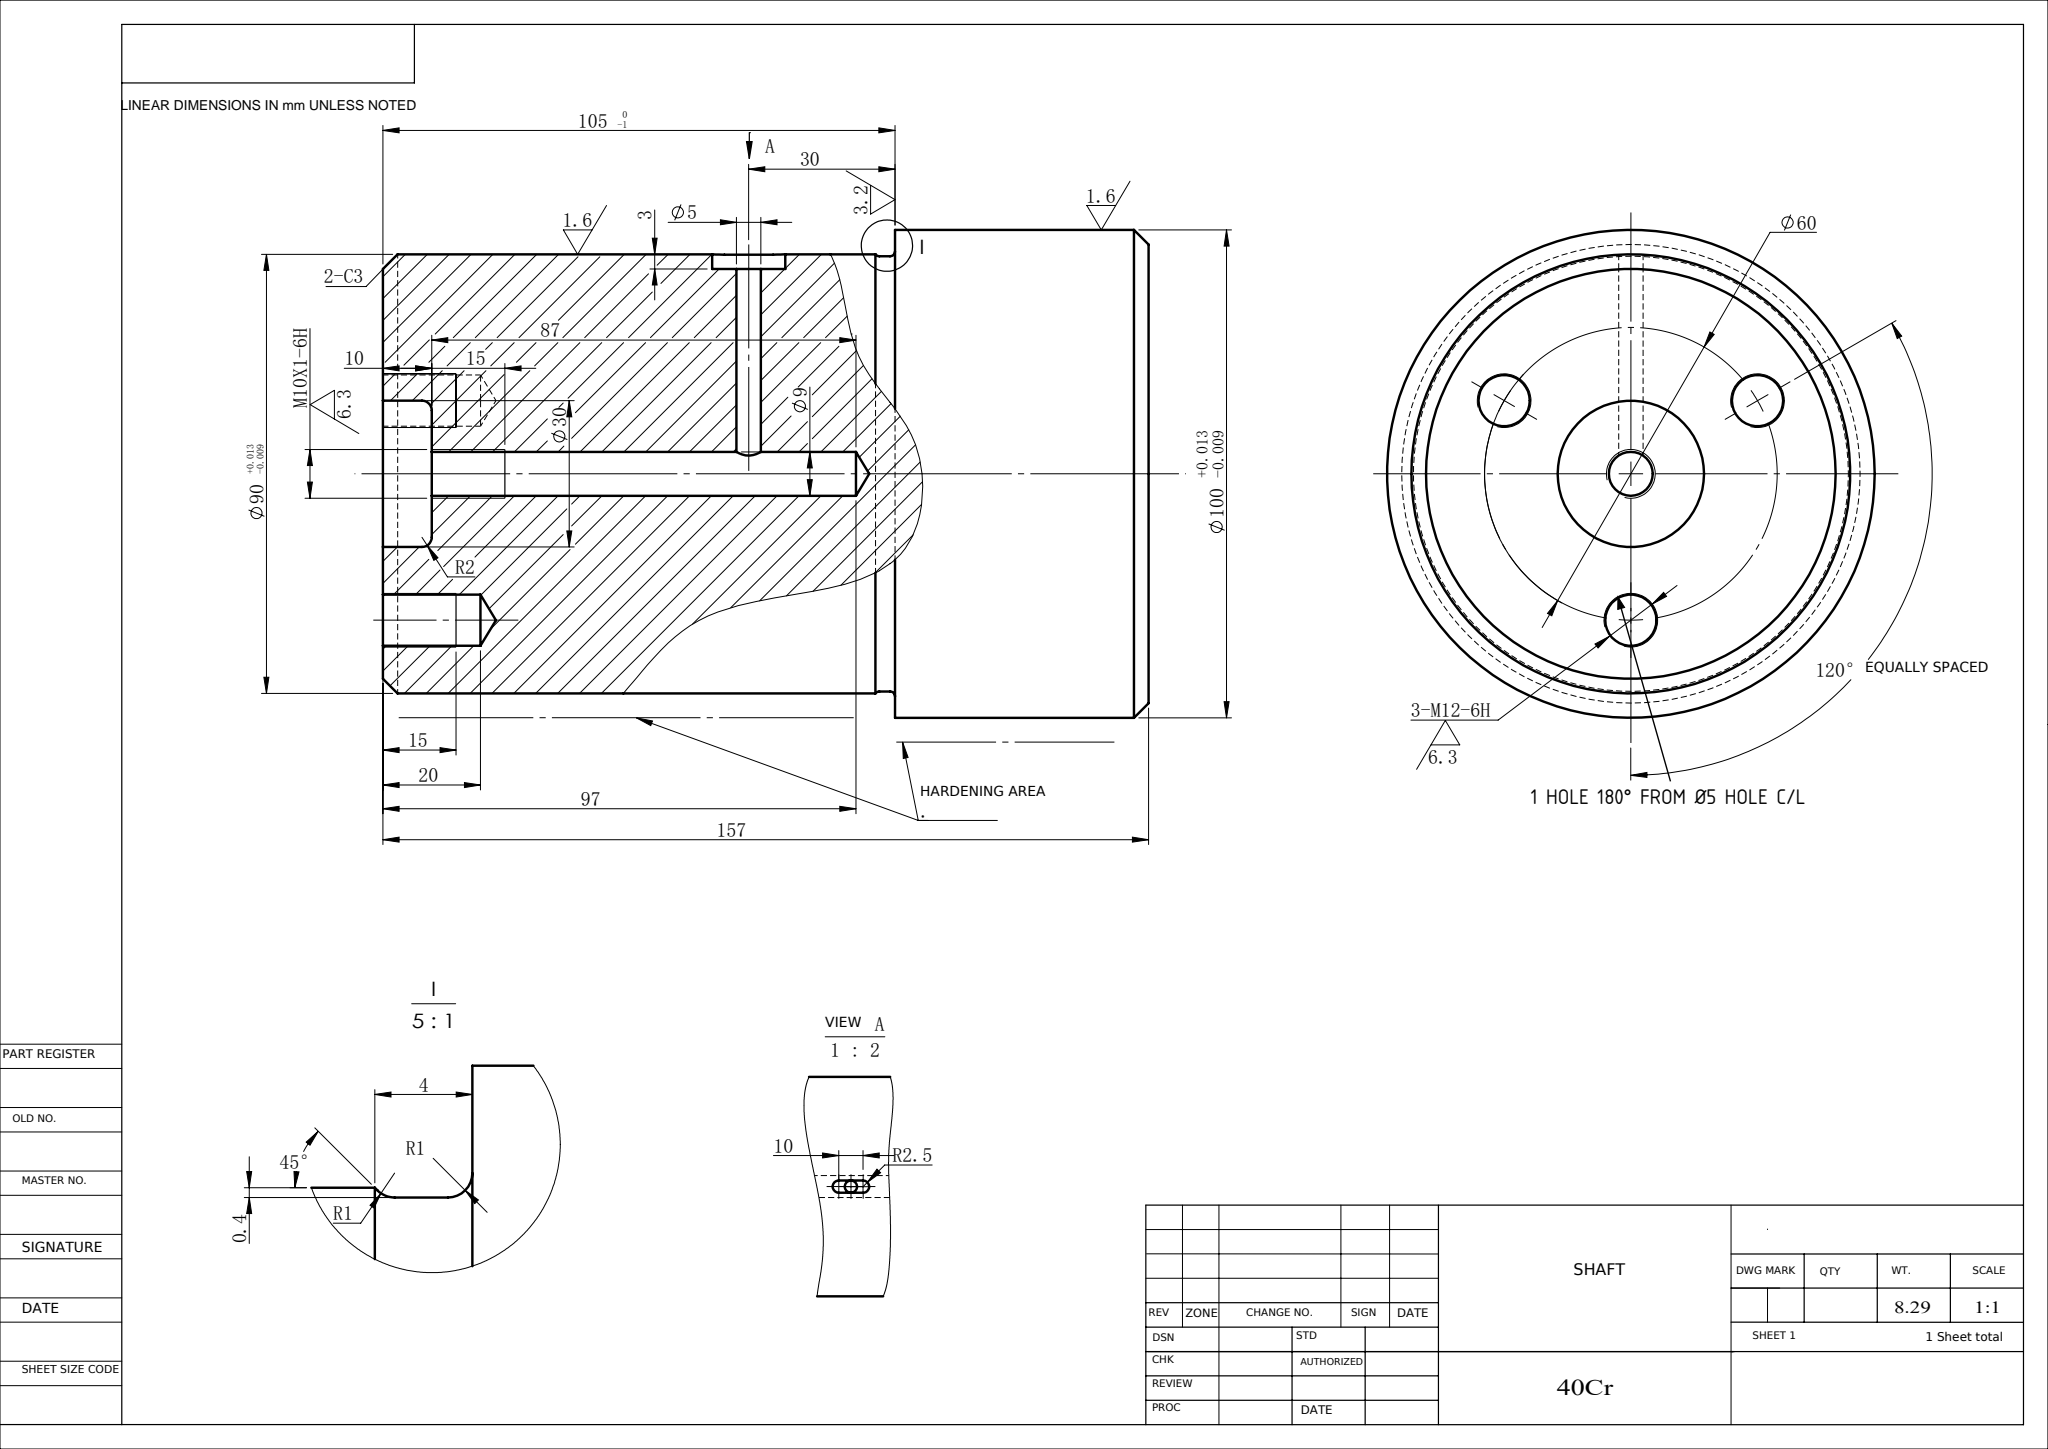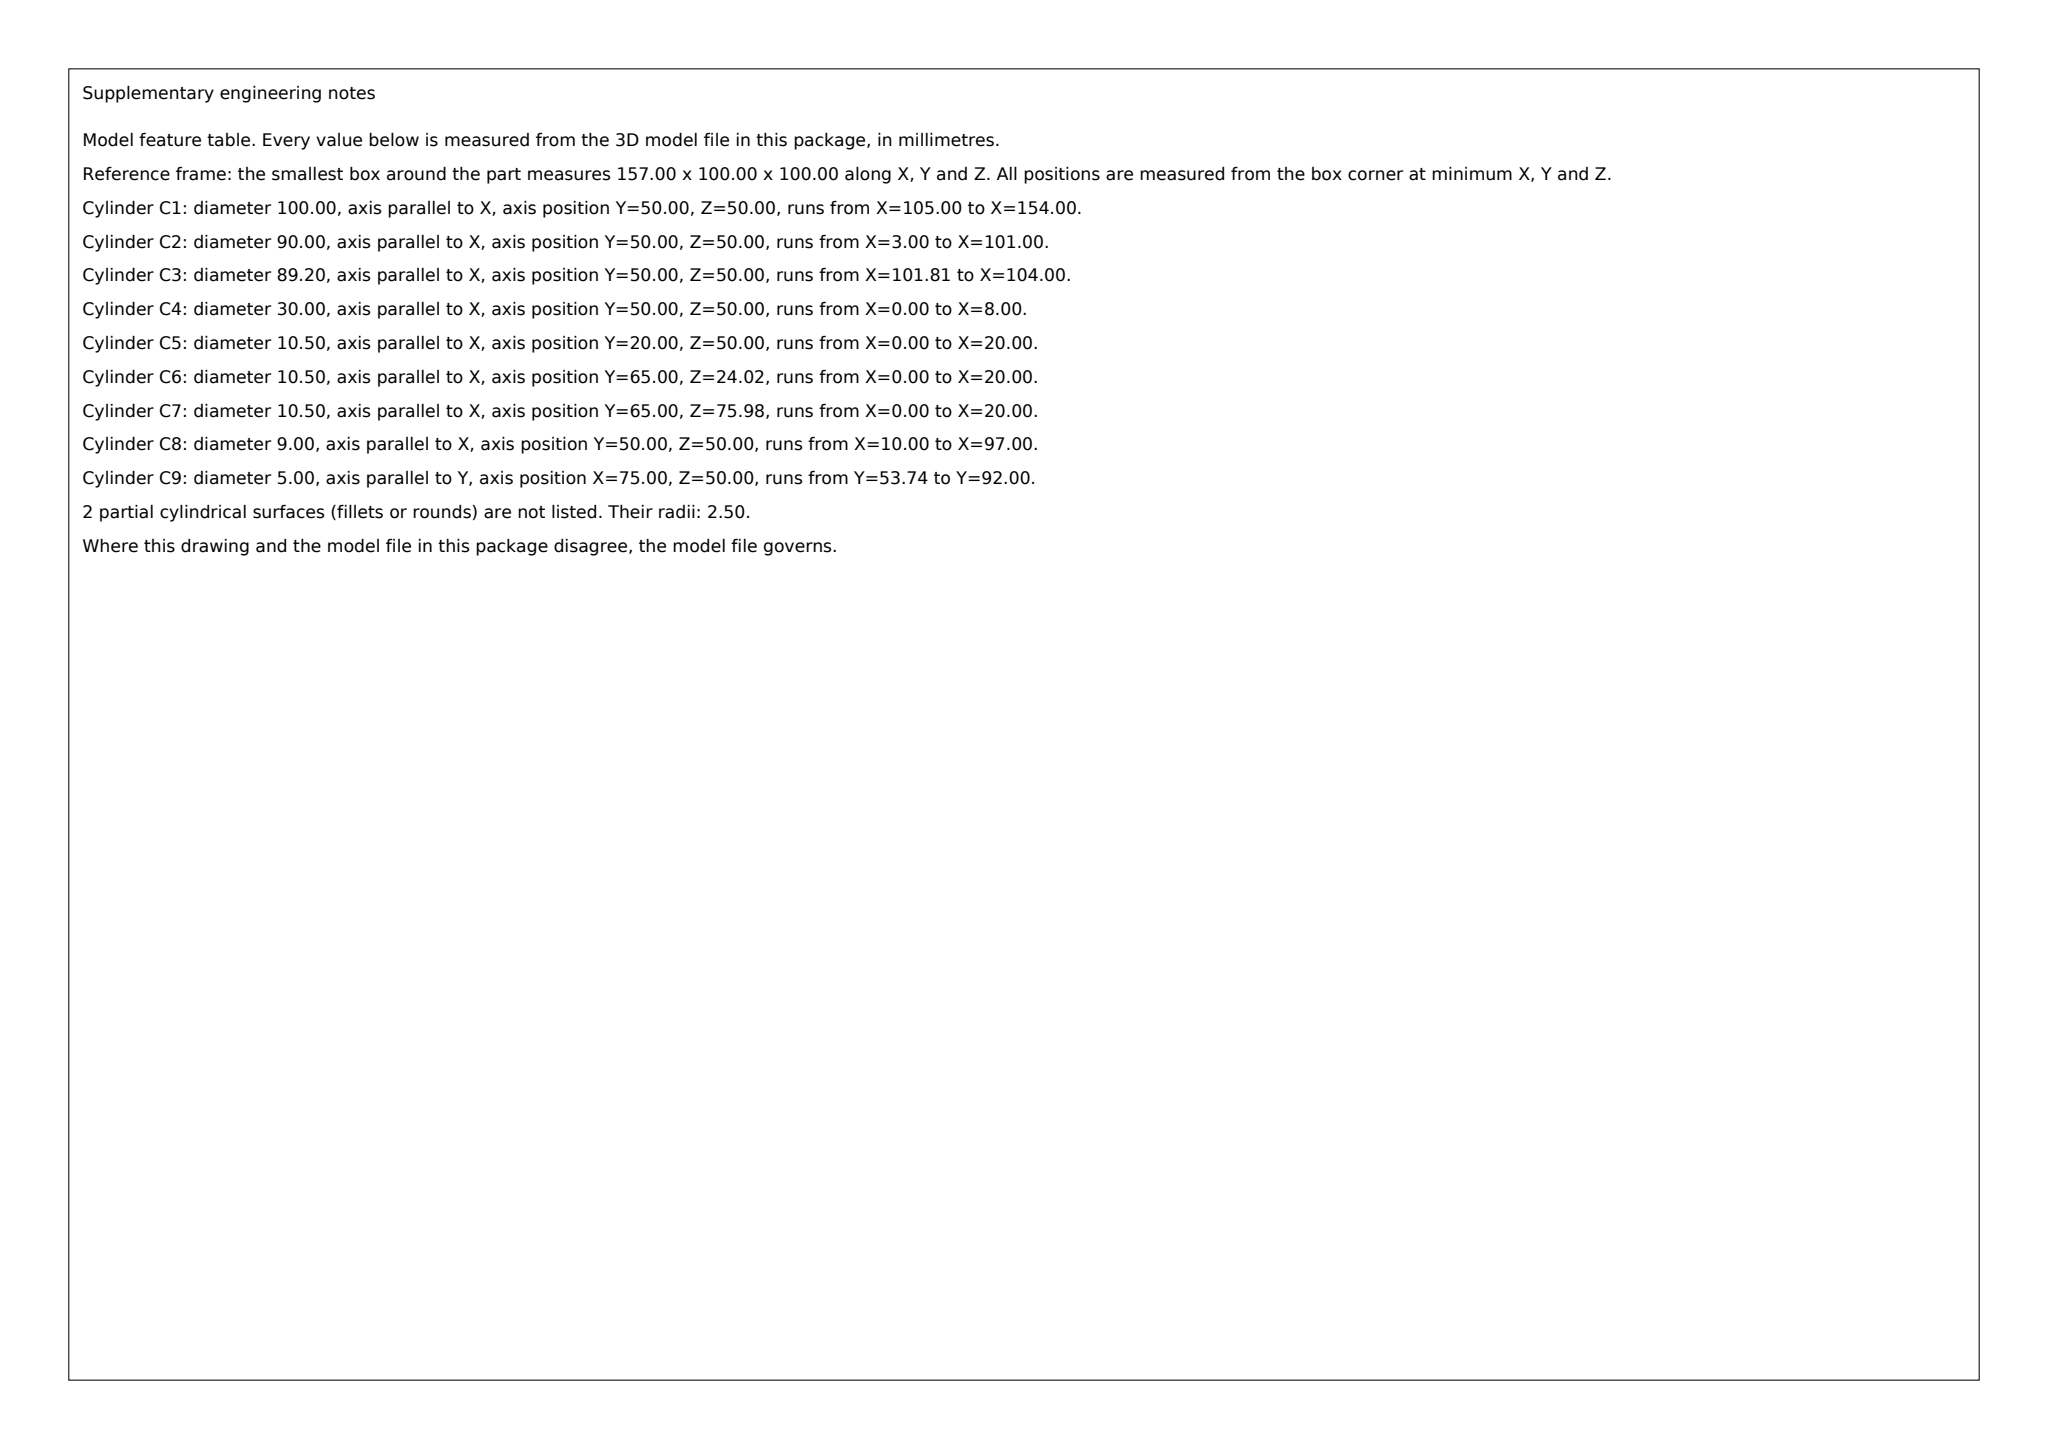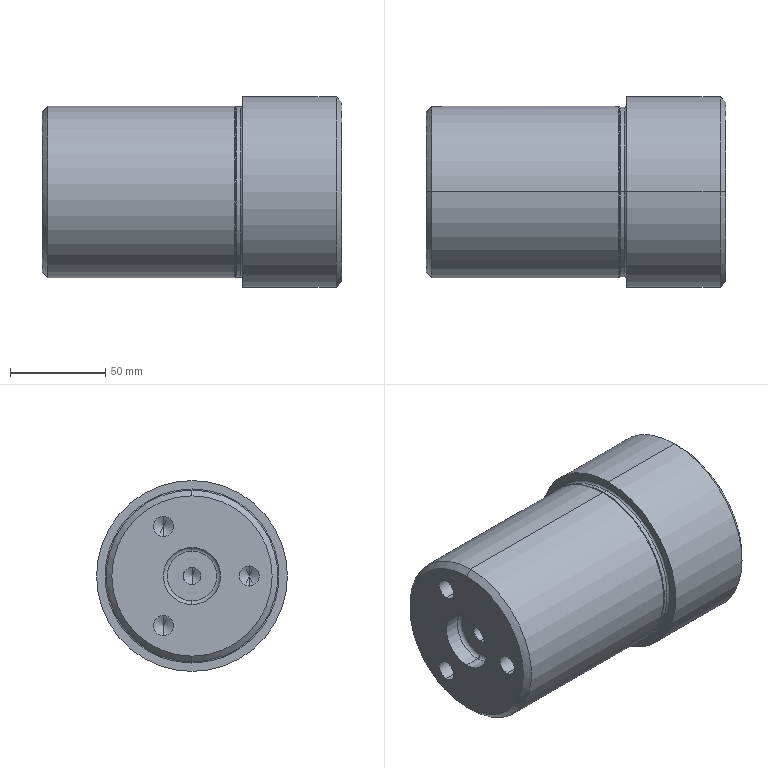Part | SolidWorks | mm | material 40Cr | 1 solid | 48 faces | box 157 x 100 x 100 mm | volume 1054399 mm3 | cylinder 20 | cone 14 | plane 8 | torus 6 | commonest cylinder face diameters 10.5 x6 5 x4 9 x2 30 x2 100 x2 89.2 x2 90 x2
Drawing notes:
3-M12-6H CLOCKING: 1 HOLE 180° FROM Ø5 CROSS HOLE C/L, OTHERS ±60° | from the solid: M12 tap drills Ø10.5 at (y,z)=(20.1,50.1),(65.1,24.1),(65.1,76.1) about axis (50.1,50.1); Ø5 cross hole axis y at z=50.1 exits +y side, so one hole lies on same C/L diametrically opposite, others at ±60° (120° equally spaced)
build123d program:
from build123d import *

# Parameters (mm, degrees)
FILLET1_R                  = 1
CHAMFER1_SIZE              = 3
SKETCH2_R                  = 15
CUT_EXTRUDE1_DEPTH         = 10
M10X1_0_TAPPED_HOLE1_D     = 9
M10X1_0_TAPPED_HOLE1_DEPTH = 87
M10X1_0_TAPPED_HOLE1_TIP   = 2.704
CUT_EXTRUDE2_DEPTH         = 3
CUT_EXTRUDE3_REACH         = 190.714
CUT_EXTRUDE3_END_RADIUS    = 4.5
SKETCH7_R                  = 2.5
FILLET2_R                  = 2
CIRPATTERN1_COUNT          = 3


with BuildPart() as part:
    # Sketch1 → Revolve1 (revolve)
    with BuildSketch(Plane.XY, mode=Mode.PRIVATE) as revolve1_sk:
        with BuildLine():
            Line((0, 0), (0, 45))
            Line((0, 45), (101, 45))
            Line((101, 45), (101.4, 44.6))
            Line((101.4, 44.6), (104, 44.6))
            ThreePointArc((104, 44.6), (104.707, 44.893), (105, 45.6))
            Line((105, 45.6), (105, 50))
            Line((105, 50), (157, 50))
            Line((157, 50), (157, 0))
            Line((157, 0), (0, 0))
        make_face()
    revolve(revolve1_sk.sketch.rotate(Axis((-80.553, 0, 0), (1, 0, 0)), 90), axis=Axis((-80.553, 0, 0), (1, 0, 0)))

    # Fillet1
    fillet1_edges = [part.edges().sort_by_distance(p)[0] for p in [
        (101.4, 0, -44.6),
    ]]
    fillet(fillet1_edges, radius=FILLET1_R)

    # Chamfer1
    chamfer1_edges = [part.edges().sort_by_distance(p)[0] for p in [
        (157, 0, -50),
        (0, 0, -45),
    ]]
    chamfer(chamfer1_edges, length=CHAMFER1_SIZE)

    # Sketch2 → Cut-Extrude1 (cut)
    with BuildSketch(Plane.ZY):
        Circle(SKETCH2_R)
    extrude(amount=-CUT_EXTRUDE1_DEPTH, mode=Mode.SUBTRACT)

    # M10x1.0 Tapped Hole1
    with Locations(Plane.ZY.offset(-10)):
        with Locations((0, 0)):
            Hole(M10X1_0_TAPPED_HOLE1_D / 2, depth=M10X1_0_TAPPED_HOLE1_DEPTH)
            with Locations((0, 0, -(M10X1_0_TAPPED_HOLE1_DEPTH + M10X1_0_TAPPED_HOLE1_TIP / 2))):  # 118° drill point
                Cone(0, M10X1_0_TAPPED_HOLE1_D / 2, M10X1_0_TAPPED_HOLE1_TIP, mode=Mode.SUBTRACT)

    # Sketch6 → Cut-Extrude2 (cut)
    with BuildSketch(Plane(origin=(0, 45, 0), x_dir=(1, 0, 0), z_dir=(0, 1, 0))):
        with BuildLine():
            Line((70, 2.5), (80, 2.5))
            ThreePointArc((80, 2.5), (82.5, 0), (80, -2.5))
            Line((80, -2.5), (70, -2.5))
            ThreePointArc((70, -2.5), (67.5, 0), (70, 2.5))
        make_face()
    extrude(amount=-CUT_EXTRUDE2_DEPTH, mode=Mode.SUBTRACT)

    # Cut-Extrude3: up to this cylinder (the profile starts outside it)
    cut_extrude3_end = Plane(origin=(75, 0, 0), z_dir=(-1, 0, 0)) * Cylinder(CUT_EXTRUDE3_END_RADIUS, 391.428, mode=Mode.PRIVATE)
    # Sketch7 → Cut-Extrude3 (cut, up to the surface)
    with BuildSketch(Plane(origin=(0, 42, 0), x_dir=(1, 0, 0), z_dir=(0, 1, 0)), mode=Mode.PRIVATE) as cut_extrude3_sk1:
        with Locations(Location((75, 0, 0), (0, 0, 270))):
            Circle(SKETCH7_R)
    cut_extrude3_tool1 = extrude(cut_extrude3_sk1.sketch, amount=-CUT_EXTRUDE3_REACH, mode=Mode.PRIVATE) - cut_extrude3_end
    add(cut_extrude3_tool1.solids().sort_by_distance((75, 42, 0))[0], mode=Mode.SUBTRACT)

    # Fillet2
    fillet2_edges = [part.edges().sort_by_distance(p)[0] for p in [
        (10, 0, -15),
    ]]
    fillet(fillet2_edges, radius=FILLET2_R)

    # Sketch8 → M12x1.5 Tapped Hole1 (revolve, cut)
    with BuildSketch(Plane.ZX.offset(-30)):
        Polygon((0, 0), (0, 23.155), (5.25, 20), (5.25, 0), align=None)
    m12x1_5_tapped_hole1 = revolve(axis=Axis((-6.35, -30, 0), (1, 0, 0)), mode=Mode.SUBTRACT)

    # CirPattern1: M12x1.5 Tapped Hole1 ×3 about axis
    cirpattern1_axis = Axis((0, 0, 0), (1, 0, 0))
    for i in range(1, CIRPATTERN1_COUNT):
        add(m12x1_5_tapped_hole1.rotate(cirpattern1_axis, i * 360 / CIRPATTERN1_COUNT), mode=Mode.SUBTRACT)


solid = part.part